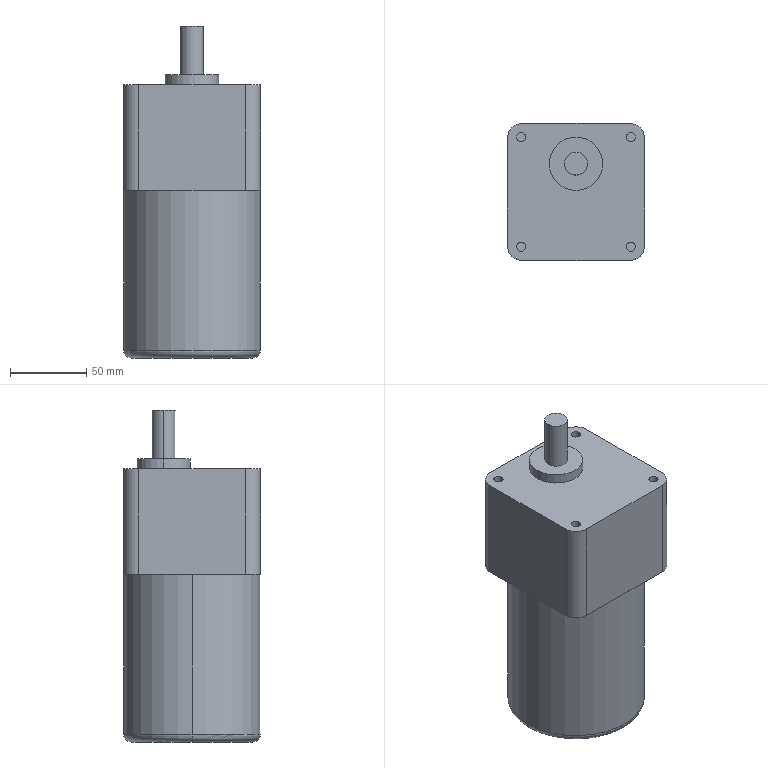Component | SolidWorks | --MA18S20041115GU-50KB90W-1 | 1 solid | 33 faces | box 90 x 90 x 218 mm | volume 1262403 mm3 | cylinder 18 | plane 13 | torus 2 | commonest cylinder face diameters 6 x8 20 x4 15 x2 35 x2 89.8 x2
build123d program:
from build123d import *

# Parameters (mm, degrees)
SKETCH1_W          = 90
SKETCH1_H          = 90
EXTRUDE1_DEPTH     = 69.5
SKETCH2_R          = 44.9
EXTRUDE2_DEPTH     = 110
SKETCH3_R          = 3
CUT_EXTRUDE1_DEPTH = 15
SKETCH4_R          = 17.5
EXTRUDE3_DEPTH     = 6.5
SKETCH5_R          = 7.5
EXTRUDE4_DEPTH     = 32
FILLET1_R          = 10
FILLET2_R          = 5


with BuildPart() as part:
    # Sketch1 → Extrude1 (new body)
    with BuildSketch(Plane.XY):
        Rectangle(SKETCH1_W, SKETCH1_H)
    extrude(amount=-EXTRUDE1_DEPTH)

    # Sketch2 → Extrude2 (add)
    with BuildSketch(Plane(origin=(0, 0, -69.5), x_dir=(-1, 0, 0), z_dir=(0, 0, -1))):
        with Locations(Location((0, 0, 0), (0, 0, 180))):
            Circle(SKETCH2_R)
    extrude(amount=EXTRUDE2_DEPTH)

    # Sketch3 → Cut-Extrude1 (cut)
    with BuildSketch(Plane.XY):
        with Locations((-36, 36)):
            Circle(SKETCH3_R)
        with Locations(Location((36, 36, 0), (0, 0, 180))):
            Circle(SKETCH3_R)
        with Locations((36, -36)):
            Circle(SKETCH3_R)
        with Locations(Location((-36, -36, 0), (0, 0, 180))):
            Circle(SKETCH3_R)
    extrude(amount=-CUT_EXTRUDE1_DEPTH, mode=Mode.SUBTRACT)

    # Sketch4 → Extrude3 (add)
    with BuildSketch(Plane.XY):
        with Locations(Location((0, 18.5, 0), (0, 0, 180))):
            Circle(SKETCH4_R)
    extrude(amount=EXTRUDE3_DEPTH)

    # Sketch5 → Extrude4 (add)
    with BuildSketch(Plane.XY.offset(6.5)):
        with Locations((0, 18.5)):
            Circle(SKETCH5_R)
    extrude(amount=EXTRUDE4_DEPTH)

    # Fillet1
    fillet1_edges = [part.edges().sort_by_distance(p)[0] for p in [
        (-45, 45, -34.75),
        (45, 45, -34.75),
        (45, -45, -34.75),
        (-45, -45, -34.75),
    ]]
    fillet(fillet1_edges, radius=FILLET1_R)

    # Fillet2
    fillet2_edges = [part.edges().sort_by_distance(p)[0] for p in [
        (-44.9, 0, -179.5),
    ]]
    fillet(fillet2_edges, radius=FILLET2_R)


solid = part.part

# Placed as in the assembly
solid = solid.moved(Location((245.885, -89.801, 61), (0, 0, 0)))
STEP:
#1=COLOUR_RGB('',0.7922,0.8196,0.9333);
#2=FILL_AREA_STYLE_COLOUR('',#1);
#3=FILL_AREA_STYLE('',(#2));
#4=SURFACE_STYLE_FILL_AREA(#3);
#5=SURFACE_SIDE_STYLE('',(#4));
#6=SURFACE_STYLE_USAGE(.BOTH.,#5);
#7=PRESENTATION_STYLE_ASSIGNMENT((#6));
#8=CARTESIAN_POINT('',(11.448,-3.535,-4.469));
#9=VERTEX_POINT('',#8);
#10=CARTESIAN_POINT('',(7.913,-3.535,-4.469));
#11=VERTEX_POINT('',#10);
#12=CARTESIAN_POINT('',(9.681,-3.535,-4.469));
#13=DIRECTION('',(0.,0.,1.));
#14=DIRECTION('',(-1.,0.,0.));
#15=AXIS2_PLACEMENT_3D('',#12,#13,#14);
#16=CIRCLE('',#15,1.768);
#17=EDGE_CURVE('',#9,#11,#16,.T.);
#18=ORIENTED_EDGE('',*,*,#17,.F.);
#19=CARTESIAN_POINT('',(11.251,-3.535,-4.665));
#20=VERTEX_POINT('',#19);
#21=CARTESIAN_POINT('',(11.251,-3.535,-4.469));
#22=DIRECTION('',(-0.,1.,0.));
#23=DIRECTION('',(-1.,0.,0.));
#24=AXIS2_PLACEMENT_3D('',#21,#22,#23);
#25=CIRCLE('',#24,0.1969);
#26=EDGE_CURVE('',#9,#20,#25,.T.);
#27=ORIENTED_EDGE('',*,*,#26,.T.);
#28=CARTESIAN_POINT('',(8.11,-3.535,-4.665));
#29=VERTEX_POINT('',#28);
#30=CARTESIAN_POINT('',(9.681,-3.535,-4.665));
#31=DIRECTION('',(0.,0.,-1.));
#32=DIRECTION('',(-1.,0.,0.));
#33=AXIS2_PLACEMENT_3D('',#30,#31,#32);
#34=CIRCLE('',#33,1.571);
#35=EDGE_CURVE('',#29,#20,#34,.T.);
#36=ORIENTED_EDGE('',*,*,#35,.F.);
#37=CARTESIAN_POINT('',(8.11,-3.535,-4.469));
#38=DIRECTION('',(0.,-1.,0.));
#39=DIRECTION('',(0.,0.,-1.));
#40=AXIS2_PLACEMENT_3D('',#37,#38,#39);
#41=CIRCLE('',#40,0.1969);
#42=EDGE_CURVE('',#11,#29,#41,.T.);
#43=ORIENTED_EDGE('',*,*,#42,.F.);
#44=EDGE_LOOP('',(#18,#27,#36,#43));
#45=FACE_OUTER_BOUND('',#44,.T.);
#46=CARTESIAN_POINT('',(9.681,-3.535,-4.469));
#47=DIRECTION('',(0.,0.,-1.));
#48=DIRECTION('',(-1.,0.,0.));
#49=AXIS2_PLACEMENT_3D('',#46,#47,#48);
#50=TOROIDAL_SURFACE('',#49,1.571,0.1969);
#51=ADVANCED_FACE('',(#45),#50,.T.);
#52=CARTESIAN_POINT('',(9.976,-2.807,3.917));
#53=VERTEX_POINT('',#52);
#54=CARTESIAN_POINT('',(9.385,-2.807,3.917));
#55=VERTEX_POINT('',#54);
#56=CARTESIAN_POINT('',(9.681,-2.807,3.917));
#57=DIRECTION('',(0.,0.,1.));
#58=DIRECTION('',(1.,0.,0.));
#59=AXIS2_PLACEMENT_3D('',#56,#57,#58);
#60=CIRCLE('',#59,0.2953);
#61=EDGE_CURVE('',#53,#55,#60,.T.);
#62=ORIENTED_EDGE('',*,*,#61,.F.);
#63=CARTESIAN_POINT('',(9.976,-2.807,2.657));
#64=VERTEX_POINT('',#63);
#65=CARTESIAN_POINT('',(9.976,-2.807,3.917));
#66=DIRECTION('',(0.,0.,-1.));
#67=VECTOR('',#66,39.37);
#68=LINE('',#65,#67);
#69=EDGE_CURVE('',#53,#64,#68,.T.);
#70=ORIENTED_EDGE('',*,*,#69,.T.);
#71=CARTESIAN_POINT('',(9.385,-2.807,2.657));
#72=VERTEX_POINT('',#71);
#73=CARTESIAN_POINT('',(9.681,-2.807,2.657));
#74=DIRECTION('',(0.,0.,1.));
#75=DIRECTION('',(1.,0.,0.));
#76=AXIS2_PLACEMENT_3D('',#73,#74,#75);
#77=CIRCLE('',#76,0.2953);
#78=EDGE_CURVE('',#64,#72,#77,.T.);
#79=ORIENTED_EDGE('',*,*,#78,.T.);
#80=CARTESIAN_POINT('',(9.385,-2.807,3.917));
#81=DIRECTION('',(0.,0.,-1.));
#82=VECTOR('',#81,39.37);
#83=LINE('',#80,#82);
#84=EDGE_CURVE('',#55,#72,#83,.T.);
#85=ORIENTED_EDGE('',*,*,#84,.F.);
#86=EDGE_LOOP('',(#62,#70,#79,#85));
#87=FACE_OUTER_BOUND('',#86,.T.);
#88=CARTESIAN_POINT('',(9.681,-2.807,3.917));
#89=DIRECTION('',(0.,0.,-1.));
#90=DIRECTION('',(-1.,0.,0.));
#91=AXIS2_PLACEMENT_3D('',#88,#89,#90);
#92=CYLINDRICAL_SURFACE('',#91,0.2953);
#93=ADVANCED_FACE('',(#87),#92,.T.);
#94=CARTESIAN_POINT('',(10.369,-2.807,2.657));
#95=VERTEX_POINT('',#94);
#96=CARTESIAN_POINT('',(8.992,-2.807,2.657));
#97=VERTEX_POINT('',#96);
#98=CARTESIAN_POINT('',(9.681,-2.807,2.657));
#99=DIRECTION('',(0.,0.,1.));
#100=DIRECTION('',(1.,0.,0.));
#101=AXIS2_PLACEMENT_3D('',#98,#99,#100);
#102=CIRCLE('',#101,0.689);
#103=EDGE_CURVE('',#95,#97,#102,.T.);
#104=ORIENTED_EDGE('',*,*,#103,.F.);
#105=CARTESIAN_POINT('',(10.369,-2.807,2.402));
#106=VERTEX_POINT('',#105);
#107=CARTESIAN_POINT('',(10.369,-2.807,2.657));
#108=DIRECTION('',(0.,0.,-1.));
#109=VECTOR('',#108,39.37);
#110=LINE('',#107,#109);
#111=EDGE_CURVE('',#95,#106,#110,.T.);
#112=ORIENTED_EDGE('',*,*,#111,.T.);
#113=CARTESIAN_POINT('',(8.992,-2.807,2.402));
#114=VERTEX_POINT('',#113);
#115=CARTESIAN_POINT('',(9.681,-2.807,2.402));
#116=DIRECTION('',(0.,0.,1.));
#117=DIRECTION('',(1.,0.,0.));
#118=AXIS2_PLACEMENT_3D('',#115,#116,#117);
#119=CIRCLE('',#118,0.689);
#120=EDGE_CURVE('',#106,#114,#119,.T.);
#121=ORIENTED_EDGE('',*,*,#120,.T.);
#122=CARTESIAN_POINT('',(8.992,-2.807,2.657));
#123=DIRECTION('',(0.,0.,-1.));
#124=VECTOR('',#123,39.37);
#125=LINE('',#122,#124);
#126=EDGE_CURVE('',#97,#114,#125,.T.);
#127=ORIENTED_EDGE('',*,*,#126,.F.);
#128=EDGE_LOOP('',(#104,#112,#121,#127));
#129=FACE_OUTER_BOUND('',#128,.T.);
#130=CARTESIAN_POINT('',(9.681,-2.807,2.657));
#131=DIRECTION('',(0.,0.,-1.));
#132=DIRECTION('',(-1.,0.,0.));
#133=AXIS2_PLACEMENT_3D('',#130,#131,#132);
#134=CYLINDRICAL_SURFACE('',#133,0.689);
#135=ADVANCED_FACE('',(#129),#134,.T.);
#136=CARTESIAN_POINT('',(8.145,-4.953,1.811));
#137=VERTEX_POINT('',#136);
#138=CARTESIAN_POINT('',(8.381,-4.953,1.811));
#139=VERTEX_POINT('',#138);
#140=CARTESIAN_POINT('',(8.263,-4.953,1.811));
#141=DIRECTION('',(0.,0.,1.));
#142=DIRECTION('',(-1.,0.,0.));
#143=AXIS2_PLACEMENT_3D('',#140,#141,#142);
#144=CIRCLE('',#143,0.1181);
#145=EDGE_CURVE('',#137,#139,#144,.T.);
#146=ORIENTED_EDGE('',*,*,#145,.F.);
#147=CARTESIAN_POINT('',(8.145,-4.953,2.402));
#148=VERTEX_POINT('',#147);
#149=CARTESIAN_POINT('',(8.145,-4.953,1.811));
#150=DIRECTION('',(0.,0.,1.));
#151=VECTOR('',#150,39.37);
#152=LINE('',#149,#151);
#153=EDGE_CURVE('',#137,#148,#152,.T.);
#154=ORIENTED_EDGE('',*,*,#153,.T.);
#155=CARTESIAN_POINT('',(8.381,-4.953,2.402));
#156=VERTEX_POINT('',#155);
#157=CARTESIAN_POINT('',(8.263,-4.953,2.402));
#158=DIRECTION('',(0.,0.,1.));
#159=DIRECTION('',(-1.,0.,0.));
#160=AXIS2_PLACEMENT_3D('',#157,#158,#159);
#161=CIRCLE('',#160,0.1181);
#162=EDGE_CURVE('',#148,#156,#161,.T.);
#163=ORIENTED_EDGE('',*,*,#162,.T.);
#164=CARTESIAN_POINT('',(8.381,-4.953,1.811));
#165=DIRECTION('',(0.,0.,1.));
#166=VECTOR('',#165,39.37);
#167=LINE('',#164,#166);
#168=EDGE_CURVE('',#139,#156,#167,.T.);
#169=ORIENTED_EDGE('',*,*,#168,.F.);
#170=EDGE_LOOP('',(#146,#154,#163,#169));
#171=FACE_OUTER_BOUND('',#170,.T.);
#172=CARTESIAN_POINT('',(8.263,-4.953,1.811));
#173=DIRECTION('',(0.,0.,1.));
#174=DIRECTION('',(1.,0.,0.));
#175=AXIS2_PLACEMENT_3D('',#172,#173,#174);
#176=CYLINDRICAL_SURFACE('',#175,0.1181);
#177=ADVANCED_FACE('',(#171),#176,.F.);
#178=CARTESIAN_POINT('',(10.98,-4.953,1.811));
#179=VERTEX_POINT('',#178);
#180=CARTESIAN_POINT('',(11.216,-4.953,1.811));
#181=VERTEX_POINT('',#180);
#182=CARTESIAN_POINT('',(11.098,-4.953,1.811));
#183=DIRECTION('',(0.,0.,1.));
#184=DIRECTION('',(1.,0.,0.));
#185=AXIS2_PLACEMENT_3D('',#182,#183,#184);
#186=CIRCLE('',#185,0.1181);
#187=EDGE_CURVE('',#179,#181,#186,.T.);
#188=ORIENTED_EDGE('',*,*,#187,.F.);
#189=CARTESIAN_POINT('',(10.98,-4.953,2.402));
#190=VERTEX_POINT('',#189);
#191=CARTESIAN_POINT('',(10.98,-4.953,1.811));
#192=DIRECTION('',(0.,0.,1.));
#193=VECTOR('',#192,39.37);
#194=LINE('',#191,#193);
#195=EDGE_CURVE('',#179,#190,#194,.T.);
#196=ORIENTED_EDGE('',*,*,#195,.T.);
#197=CARTESIAN_POINT('',(11.216,-4.953,2.402));
#198=VERTEX_POINT('',#197);
#199=CARTESIAN_POINT('',(11.098,-4.953,2.402));
#200=DIRECTION('',(0.,0.,1.));
#201=DIRECTION('',(1.,0.,0.));
#202=AXIS2_PLACEMENT_3D('',#199,#200,#201);
#203=CIRCLE('',#202,0.1181);
#204=EDGE_CURVE('',#190,#198,#203,.T.);
#205=ORIENTED_EDGE('',*,*,#204,.T.);
#206=CARTESIAN_POINT('',(11.216,-4.953,1.811));
#207=DIRECTION('',(0.,0.,1.));
#208=VECTOR('',#207,39.37);
#209=LINE('',#206,#208);
#210=EDGE_CURVE('',#181,#198,#209,.T.);
#211=ORIENTED_EDGE('',*,*,#210,.F.);
#212=EDGE_LOOP('',(#188,#196,#205,#211));
#213=FACE_OUTER_BOUND('',#212,.T.);
#214=CARTESIAN_POINT('',(11.098,-4.953,1.811));
#215=DIRECTION('',(0.,0.,1.));
#216=DIRECTION('',(1.,0.,0.));
#217=AXIS2_PLACEMENT_3D('',#214,#215,#216);
#218=CYLINDRICAL_SURFACE('',#217,0.1181);
#219=ADVANCED_FACE('',(#213),#218,.F.);
#220=CARTESIAN_POINT('',(10.98,-2.118,1.811));
#221=VERTEX_POINT('',#220);
#222=CARTESIAN_POINT('',(11.216,-2.118,1.811));
#223=VERTEX_POINT('',#222);
#224=CARTESIAN_POINT('',(11.098,-2.118,1.811));
#225=DIRECTION('',(0.,0.,1.));
#226=DIRECTION('',(-1.,0.,0.));
#227=AXIS2_PLACEMENT_3D('',#224,#225,#226);
#228=CIRCLE('',#227,0.1181);
#229=EDGE_CURVE('',#221,#223,#228,.T.);
#230=ORIENTED_EDGE('',*,*,#229,.F.);
#231=CARTESIAN_POINT('',(10.98,-2.118,2.402));
#232=VERTEX_POINT('',#231);
#233=CARTESIAN_POINT('',(10.98,-2.118,1.811));
#234=DIRECTION('',(0.,0.,1.));
#235=VECTOR('',#234,39.37);
#236=LINE('',#233,#235);
#237=EDGE_CURVE('',#221,#232,#236,.T.);
#238=ORIENTED_EDGE('',*,*,#237,.T.);
#239=CARTESIAN_POINT('',(11.216,-2.118,2.402));
#240=VERTEX_POINT('',#239);
#241=CARTESIAN_POINT('',(11.098,-2.118,2.402));
#242=DIRECTION('',(0.,0.,1.));
#243=DIRECTION('',(-1.,0.,0.));
#244=AXIS2_PLACEMENT_3D('',#241,#242,#243);
#245=CIRCLE('',#244,0.1181);
#246=EDGE_CURVE('',#232,#240,#245,.T.);
#247=ORIENTED_EDGE('',*,*,#246,.T.);
#248=CARTESIAN_POINT('',(11.216,-2.118,1.811));
#249=DIRECTION('',(0.,0.,1.));
#250=VECTOR('',#249,39.37);
#251=LINE('',#248,#250);
#252=EDGE_CURVE('',#223,#240,#251,.T.);
#253=ORIENTED_EDGE('',*,*,#252,.F.);
#254=EDGE_LOOP('',(#230,#238,#247,#253));
#255=FACE_OUTER_BOUND('',#254,.T.);
#256=CARTESIAN_POINT('',(11.098,-2.118,1.811));
#257=DIRECTION('',(0.,0.,1.));
#258=DIRECTION('',(1.,0.,0.));
#259=AXIS2_PLACEMENT_3D('',#256,#257,#258);
#260=CYLINDRICAL_SURFACE('',#259,0.1181);
#261=ADVANCED_FACE('',(#255),#260,.F.);
#262=CARTESIAN_POINT('',(8.145,-2.118,1.811));
#263=VERTEX_POINT('',#262);
#264=CARTESIAN_POINT('',(8.381,-2.118,1.811));
#265=VERTEX_POINT('',#264);
#266=CARTESIAN_POINT('',(8.263,-2.118,1.811));
#267=DIRECTION('',(0.,0.,1.));
#268=DIRECTION('',(1.,0.,0.));
#269=AXIS2_PLACEMENT_3D('',#266,#267,#268);
#270=CIRCLE('',#269,0.1181);
#271=EDGE_CURVE('',#263,#265,#270,.T.);
#272=ORIENTED_EDGE('',*,*,#271,.F.);
#273=CARTESIAN_POINT('',(8.145,-2.118,2.402));
#274=VERTEX_POINT('',#273);
#275=CARTESIAN_POINT('',(8.145,-2.118,1.811));
#276=DIRECTION('',(0.,0.,1.));
#277=VECTOR('',#276,39.37);
#278=LINE('',#275,#277);
#279=EDGE_CURVE('',#263,#274,#278,.T.);
#280=ORIENTED_EDGE('',*,*,#279,.T.);
#281=CARTESIAN_POINT('',(8.381,-2.118,2.402));
#282=VERTEX_POINT('',#281);
#283=CARTESIAN_POINT('',(8.263,-2.118,2.402));
#284=DIRECTION('',(0.,0.,1.));
#285=DIRECTION('',(1.,0.,0.));
#286=AXIS2_PLACEMENT_3D('',#283,#284,#285);
#287=CIRCLE('',#286,0.1181);
#288=EDGE_CURVE('',#274,#282,#287,.T.);
#289=ORIENTED_EDGE('',*,*,#288,.T.);
#290=CARTESIAN_POINT('',(8.381,-2.118,1.811));
#291=DIRECTION('',(0.,0.,1.));
#292=VECTOR('',#291,39.37);
#293=LINE('',#290,#292);
#294=EDGE_CURVE('',#265,#282,#293,.T.);
#295=ORIENTED_EDGE('',*,*,#294,.F.);
#296=EDGE_LOOP('',(#272,#280,#289,#295));
#297=FACE_OUTER_BOUND('',#296,.T.);
#298=CARTESIAN_POINT('',(8.263,-2.118,1.811));
#299=DIRECTION('',(0.,0.,1.));
#300=DIRECTION('',(1.,0.,0.));
#301=AXIS2_PLACEMENT_3D('',#298,#299,#300);
#302=CYLINDRICAL_SURFACE('',#301,0.1181);
#303=ADVANCED_FACE('',(#297),#302,.F.);
#304=ORIENTED_EDGE('',*,*,#17,.T.);
#305=CARTESIAN_POINT('',(7.913,-3.535,-0.3346));
#306=VERTEX_POINT('',#305);
#307=CARTESIAN_POINT('',(7.913,-3.535,-4.665));
#308=DIRECTION('',(0.,0.,1.));
#309=VECTOR('',#308,39.37);
#310=LINE('',#307,#309);
#311=EDGE_CURVE('',#11,#306,#310,.T.);
#312=ORIENTED_EDGE('',*,*,#311,.T.);
#313=CARTESIAN_POINT('',(11.448,-3.535,-0.3346));
#314=VERTEX_POINT('',#313);
#315=CARTESIAN_POINT('',(9.681,-3.535,-0.3346));
#316=DIRECTION('',(0.,0.,-1.));
#317=DIRECTION('',(1.,0.,0.));
#318=AXIS2_PLACEMENT_3D('',#315,#316,#317);
#319=CIRCLE('',#318,1.768);
#320=EDGE_CURVE('',#306,#314,#319,.T.);
#321=ORIENTED_EDGE('',*,*,#320,.T.);
#322=CARTESIAN_POINT('',(11.448,-3.535,-4.665));
#323=DIRECTION('',(0.,0.,1.));
#324=VECTOR('',#323,39.37);
#325=LINE('',#322,#324);
#326=EDGE_CURVE('',#9,#314,#325,.T.);
#327=ORIENTED_EDGE('',*,*,#326,.F.);
#328=EDGE_LOOP('',(#304,#312,#321,#327));
#329=FACE_OUTER_BOUND('',#328,.T.);
#330=CARTESIAN_POINT('',(9.681,-3.535,-4.665));
#331=DIRECTION('',(0.,0.,1.));
#332=DIRECTION('',(1.,0.,0.));
#333=AXIS2_PLACEMENT_3D('',#330,#331,#332);
#334=CYLINDRICAL_SURFACE('',#333,1.768);
#335=ADVANCED_FACE('',(#329),#334,.T.);
#336=CARTESIAN_POINT('',(9.681,-2.807,2.657));
#337=DIRECTION('',(0.,0.,1.));
#338=DIRECTION('',(1.,0.,0.));
#339=AXIS2_PLACEMENT_3D('',#336,#337,#338);
#340=CIRCLE('',#339,0.689);
#341=EDGE_CURVE('',#97,#95,#340,.T.);
#342=ORIENTED_EDGE('',*,*,#341,.T.);
#343=ORIENTED_EDGE('',*,*,#103,.T.);
#344=EDGE_LOOP('',(#342,#343));
#345=FACE_OUTER_BOUND('',#344,.T.);
#346=CARTESIAN_POINT('',(9.681,-2.807,2.657));
#347=DIRECTION('',(0.,0.,1.));
#348=DIRECTION('',(1.,0.,0.));
#349=AXIS2_PLACEMENT_3D('',#346,#347,#348);
#350=CIRCLE('',#349,0.2953);
#351=EDGE_CURVE('',#72,#64,#350,.T.);
#352=ORIENTED_EDGE('',*,*,#351,.F.);
#353=ORIENTED_EDGE('',*,*,#78,.F.);
#354=EDGE_LOOP('',(#352,#353));
#355=FACE_BOUND('',#354,.T.);
#356=CARTESIAN_POINT('',(9.681,-2.807,2.657));
#357=DIRECTION('',(0.,0.,1.));
#358=DIRECTION('',(1.,0.,0.));
#359=AXIS2_PLACEMENT_3D('',#356,#357,#358);
#360=PLANE('',#359);
#361=ADVANCED_FACE('',(#345,#355),#360,.T.);
#362=CARTESIAN_POINT('',(7.909,-2.158,2.402));
#363=VERTEX_POINT('',#362);
#364=CARTESIAN_POINT('',(7.909,-4.913,2.402));
#365=VERTEX_POINT('',#364);
#366=CARTESIAN_POINT('',(7.909,-1.764,2.402));
#367=DIRECTION('',(0.,-1.,0.));
#368=VECTOR('',#367,39.37);
#369=LINE('',#366,#368);
#370=EDGE_CURVE('',#363,#365,#369,.T.);
#371=ORIENTED_EDGE('',*,*,#370,.T.);
#372=CARTESIAN_POINT('',(8.303,-5.307,2.402));
#373=VERTEX_POINT('',#372);
#374=CARTESIAN_POINT('',(8.303,-4.913,2.402));
#375=DIRECTION('',(0.,0.,1.));
#376=DIRECTION('',(1.,0.,0.));
#377=AXIS2_PLACEMENT_3D('',#374,#375,#376);
#378=CIRCLE('',#377,0.3937);
#379=EDGE_CURVE('',#365,#373,#378,.T.);
#380=ORIENTED_EDGE('',*,*,#379,.T.);
#381=CARTESIAN_POINT('',(11.058,-5.307,2.402));
#382=VERTEX_POINT('',#381);
#383=CARTESIAN_POINT('',(7.909,-5.307,2.402));
#384=DIRECTION('',(1.,0.,0.));
#385=VECTOR('',#384,39.37);
#386=LINE('',#383,#385);
#387=EDGE_CURVE('',#373,#382,#386,.T.);
#388=ORIENTED_EDGE('',*,*,#387,.T.);
#389=CARTESIAN_POINT('',(11.452,-4.913,2.402));
#390=VERTEX_POINT('',#389);
#391=CARTESIAN_POINT('',(11.058,-4.913,2.402));
#392=DIRECTION('',(0.,0.,1.));
#393=DIRECTION('',(1.,0.,0.));
#394=AXIS2_PLACEMENT_3D('',#391,#392,#393);
#395=CIRCLE('',#394,0.3937);
#396=EDGE_CURVE('',#382,#390,#395,.T.);
#397=ORIENTED_EDGE('',*,*,#396,.T.);
#398=CARTESIAN_POINT('',(11.452,-2.158,2.402));
#399=VERTEX_POINT('',#398);
#400=CARTESIAN_POINT('',(11.452,-1.764,2.402));
#401=DIRECTION('',(-0.,1.,0.));
#402=VECTOR('',#401,39.37);
#403=LINE('',#400,#402);
#404=EDGE_CURVE('',#390,#399,#403,.T.);
#405=ORIENTED_EDGE('',*,*,#404,.T.);
#406=CARTESIAN_POINT('',(11.058,-1.764,2.402));
#407=VERTEX_POINT('',#406);
#408=CARTESIAN_POINT('',(11.058,-2.158,2.402));
#409=DIRECTION('',(0.,0.,1.));
#410=DIRECTION('',(1.,0.,0.));
#411=AXIS2_PLACEMENT_3D('',#408,#409,#410);
#412=CIRCLE('',#411,0.3937);
#413=EDGE_CURVE('',#399,#407,#412,.T.);
#414=ORIENTED_EDGE('',*,*,#413,.T.);
#415=CARTESIAN_POINT('',(8.303,-1.764,2.402));
#416=VERTEX_POINT('',#415);
#417=CARTESIAN_POINT('',(7.909,-1.764,2.402));
#418=DIRECTION('',(-1.,-0.,0.));
#419=VECTOR('',#418,39.37);
#420=LINE('',#417,#419);
#421=EDGE_CURVE('',#407,#416,#420,.T.);
#422=ORIENTED_EDGE('',*,*,#421,.T.);
#423=CARTESIAN_POINT('',(8.303,-2.158,2.402));
#424=DIRECTION('',(0.,0.,1.));
#425=DIRECTION('',(1.,0.,0.));
#426=AXIS2_PLACEMENT_3D('',#423,#424,#425);
#427=CIRCLE('',#426,0.3937);
#428=EDGE_CURVE('',#416,#363,#427,.T.);
#429=ORIENTED_EDGE('',*,*,#428,.T.);
#430=EDGE_LOOP('',(#371,#380,#388,#397,#405,#414,#422,#429));
#431=FACE_OUTER_BOUND('',#430,.T.);
#432=CARTESIAN_POINT('',(8.263,-2.118,2.402));
#433=DIRECTION('',(0.,0.,1.));
#434=DIRECTION('',(1.,0.,0.));
#435=AXIS2_PLACEMENT_3D('',#432,#433,#434);
#436=CIRCLE('',#435,0.1181);
#437=EDGE_CURVE('',#282,#274,#436,.T.);
#438=ORIENTED_EDGE('',*,*,#437,.F.);
#439=ORIENTED_EDGE('',*,*,#288,.F.);
#440=EDGE_LOOP('',(#438,#439));
#441=FACE_BOUND('',#440,.T.);
#442=CARTESIAN_POINT('',(11.098,-2.118,2.402));
#443=DIRECTION('',(0.,0.,1.));
#444=DIRECTION('',(-1.,0.,0.));
#445=AXIS2_PLACEMENT_3D('',#442,#443,#444);
#446=CIRCLE('',#445,0.1181);
#447=EDGE_CURVE('',#240,#232,#446,.T.);
#448=ORIENTED_EDGE('',*,*,#447,.F.);
#449=ORIENTED_EDGE('',*,*,#246,.F.);
#450=EDGE_LOOP('',(#448,#449));
#451=FACE_BOUND('',#450,.T.);
#452=CARTESIAN_POINT('',(11.098,-4.953,2.402));
#453=DIRECTION('',(0.,0.,1.));
#454=DIRECTION('',(1.,0.,0.));
#455=AXIS2_PLACEMENT_3D('',#452,#453,#454);
#456=CIRCLE('',#455,0.1181);
#457=EDGE_CURVE('',#198,#190,#456,.T.);
#458=ORIENTED_EDGE('',*,*,#457,.F.);
#459=ORIENTED_EDGE('',*,*,#204,.F.);
#460=EDGE_LOOP('',(#458,#459));
#461=FACE_BOUND('',#460,.T.);
#462=CARTESIAN_POINT('',(8.263,-4.953,2.402));
#463=DIRECTION('',(0.,0.,1.));
#464=DIRECTION('',(-1.,0.,0.));
#465=AXIS2_PLACEMENT_3D('',#462,#463,#464);
#466=CIRCLE('',#465,0.1181);
#467=EDGE_CURVE('',#156,#148,#466,.T.);
#468=ORIENTED_EDGE('',*,*,#467,.F.);
#469=ORIENTED_EDGE('',*,*,#162,.F.);
#470=EDGE_LOOP('',(#468,#469));
#471=FACE_BOUND('',#470,.T.);
#472=CARTESIAN_POINT('',(9.681,-2.807,2.402));
#473=DIRECTION('',(0.,0.,1.));
#474=DIRECTION('',(1.,0.,0.));
#475=AXIS2_PLACEMENT_3D('',#472,#473,#474);
#476=CIRCLE('',#475,0.689);
#477=EDGE_CURVE('',#114,#106,#476,.T.);
#478=ORIENTED_EDGE('',*,*,#477,.F.);
#479=ORIENTED_EDGE('',*,*,#120,.F.);
#480=EDGE_LOOP('',(#478,#479));
#481=FACE_BOUND('',#480,.T.);
#482=CARTESIAN_POINT('',(7.909,-5.307,2.402));
#483=DIRECTION('',(0.,0.,1.));
#484=DIRECTION('',(1.,0.,0.));
#485=AXIS2_PLACEMENT_3D('',#482,#483,#484);
#486=PLANE('',#485);
#487=ADVANCED_FACE('',(#431,#441,#451,#461,#471,#481),#486,.T.);
#488=CARTESIAN_POINT('',(8.303,-5.307,-0.3346));
#489=VERTEX_POINT('',#488);
#490=CARTESIAN_POINT('',(11.058,-5.307,-0.3346));
#491=VERTEX_POINT('',#490);
#492=CARTESIAN_POINT('',(7.909,-5.307,-0.3346));
#493=DIRECTION('',(1.,0.,0.));
#494=VECTOR('',#493,39.37);
#495=LINE('',#492,#494);
#496=EDGE_CURVE('',#489,#491,#495,.T.);
#497=ORIENTED_EDGE('',*,*,#496,.F.);
#498=CARTESIAN_POINT('',(7.909,-4.913,-0.3346));
#499=VERTEX_POINT('',#498);
#500=CARTESIAN_POINT('',(8.303,-4.913,-0.3346));
#501=DIRECTION('',(0.,0.,-1.));
#502=DIRECTION('',(1.,0.,0.));
#503=AXIS2_PLACEMENT_3D('',#500,#501,#502);
#504=CIRCLE('',#503,0.3937);
#505=EDGE_CURVE('',#489,#499,#504,.T.);
#506=ORIENTED_EDGE('',*,*,#505,.T.);
#507=CARTESIAN_POINT('',(7.909,-2.158,-0.3346));
#508=VERTEX_POINT('',#507);
#509=CARTESIAN_POINT('',(7.909,-1.764,-0.3346));
#510=DIRECTION('',(0.,-1.,0.));
#511=VECTOR('',#510,39.37);
#512=LINE('',#509,#511);
#513=EDGE_CURVE('',#508,#499,#512,.T.);
#514=ORIENTED_EDGE('',*,*,#513,.F.);
#515=CARTESIAN_POINT('',(8.303,-1.764,-0.3346));
#516=VERTEX_POINT('',#515);
#517=CARTESIAN_POINT('',(8.303,-2.158,-0.3346));
#518=DIRECTION('',(0.,0.,-1.));
#519=DIRECTION('',(1.,0.,0.));
#520=AXIS2_PLACEMENT_3D('',#517,#518,#519);
#521=CIRCLE('',#520,0.3937);
#522=EDGE_CURVE('',#508,#516,#521,.T.);
#523=ORIENTED_EDGE('',*,*,#522,.T.);
#524=CARTESIAN_POINT('',(11.058,-1.764,-0.3346));
#525=VERTEX_POINT('',#524);
#526=CARTESIAN_POINT('',(7.909,-1.764,-0.3346));
#527=DIRECTION('',(-1.,-0.,0.));
#528=VECTOR('',#527,39.37);
#529=LINE('',#526,#528);
#530=EDGE_CURVE('',#525,#516,#529,.T.);
#531=ORIENTED_EDGE('',*,*,#530,.F.);
#532=CARTESIAN_POINT('',(11.452,-2.158,-0.3346));
#533=VERTEX_POINT('',#532);
#534=CARTESIAN_POINT('',(11.058,-2.158,-0.3346));
#535=DIRECTION('',(0.,0.,-1.));
#536=DIRECTION('',(1.,0.,0.));
#537=AXIS2_PLACEMENT_3D('',#534,#535,#536);
#538=CIRCLE('',#537,0.3937);
#539=EDGE_CURVE('',#525,#533,#538,.T.);
#540=ORIENTED_EDGE('',*,*,#539,.T.);
#541=CARTESIAN_POINT('',(11.452,-4.913,-0.3346));
#542=VERTEX_POINT('',#541);
#543=CARTESIAN_POINT('',(11.452,-1.764,-0.3346));
#544=DIRECTION('',(-0.,1.,0.));
#545=VECTOR('',#544,39.37);
#546=LINE('',#543,#545);
#547=EDGE_CURVE('',#542,#533,#546,.T.);
#548=ORIENTED_EDGE('',*,*,#547,.F.);
#549=CARTESIAN_POINT('',(11.058,-4.913,-0.3346));
#550=DIRECTION('',(0.,0.,-1.));
#551=DIRECTION('',(1.,0.,0.));
#552=AXIS2_PLACEMENT_3D('',#549,#550,#551);
#553=CIRCLE('',#552,0.3937);
#554=EDGE_CURVE('',#542,#491,#553,.T.);
#555=ORIENTED_EDGE('',*,*,#554,.T.);
#556=EDGE_LOOP('',(#497,#506,#514,#523,#531,#540,#548,#555));
#557=FACE_OUTER_BOUND('',#556,.T.);
#558=CARTESIAN_POINT('',(9.681,-3.535,-0.3346));
#559=DIRECTION('',(0.,0.,-1.));
#560=DIRECTION('',(1.,0.,0.));
#561=AXIS2_PLACEMENT_3D('',#558,#559,#560);
#562=CIRCLE('',#561,1.768);
#563=EDGE_CURVE('',#314,#306,#562,.T.);
#564=ORIENTED_EDGE('',*,*,#563,.F.);
#565=ORIENTED_EDGE('',*,*,#320,.F.);
#566=EDGE_LOOP('',(#564,#565));
#567=FACE_BOUND('',#566,.T.);
#568=CARTESIAN_POINT('',(7.909,-5.307,-0.3346));
#569=DIRECTION('',(0.,0.,1.));
#570=DIRECTION('',(1.,0.,0.));
#571=AXIS2_PLACEMENT_3D('',#568,#569,#570);
#572=PLANE('',#571);
#573=ADVANCED_FACE('',(#557,#567),#572,.F.);
#574=ORIENTED_EDGE('',*,*,#513,.T.);
#575=CARTESIAN_POINT('',(7.909,-4.913,-0.3346));
#576=DIRECTION('',(0.,0.,1.));
#577=VECTOR('',#576,39.37);
#578=LINE('',#575,#577);
#579=EDGE_CURVE('',#499,#365,#578,.T.);
#580=ORIENTED_EDGE('',*,*,#579,.T.);
#581=ORIENTED_EDGE('',*,*,#370,.F.);
#582=CARTESIAN_POINT('',(7.909,-2.158,-0.3346));
#583=DIRECTION('',(0.,0.,-1.));
#584=VECTOR('',#583,39.37);
#585=LINE('',#582,#584);
#586=EDGE_CURVE('',#363,#508,#585,.T.);
#587=ORIENTED_EDGE('',*,*,#586,.T.);
#588=EDGE_LOOP('',(#574,#580,#581,#587));
#589=FACE_OUTER_BOUND('',#588,.T.);
#590=CARTESIAN_POINT('',(7.909,-1.764,-0.3346));
#591=DIRECTION('',(-1.,-0.,0.));
#592=DIRECTION('',(0.,-1.,0.));
#593=AXIS2_PLACEMENT_3D('',#590,#591,#592);
#594=PLANE('',#593);
#595=ADVANCED_FACE('',(#589),#594,.T.);
#596=ORIENTED_EDGE('',*,*,#530,.T.);
#597=CARTESIAN_POINT('',(8.303,-1.764,-0.3346));
#598=DIRECTION('',(0.,0.,1.));
#599=VECTOR('',#598,39.37);
#600=LINE('',#597,#599);
#601=EDGE_CURVE('',#516,#416,#600,.T.);
#602=ORIENTED_EDGE('',*,*,#601,.T.);
#603=ORIENTED_EDGE('',*,*,#421,.F.);
#604=CARTESIAN_POINT('',(11.058,-1.764,-0.3346));
#605=DIRECTION('',(0.,0.,-1.));
#606=VECTOR('',#605,39.37);
#607=LINE('',#604,#606);
#608=EDGE_CURVE('',#407,#525,#607,.T.);
#609=ORIENTED_EDGE('',*,*,#608,.T.);
#610=EDGE_LOOP('',(#596,#602,#603,#609));
#611=FACE_OUTER_BOUND('',#610,.T.);
#612=CARTESIAN_POINT('',(7.909,-1.764,-0.3346));
#613=DIRECTION('',(-0.,1.,0.));
#614=DIRECTION('',(-1.,-0.,0.));
#615=AXIS2_PLACEMENT_3D('',#612,#613,#614);
#616=PLANE('',#615);
#617=ADVANCED_FACE('',(#611),#616,.T.);
#618=ORIENTED_EDGE('',*,*,#404,.F.);
#619=CARTESIAN_POINT('',(11.452,-4.913,-0.3346));
#620=DIRECTION('',(0.,0.,-1.));
#621=VECTOR('',#620,39.37);
#622=LINE('',#619,#621);
#623=EDGE_CURVE('',#390,#542,#622,.T.);
#624=ORIENTED_EDGE('',*,*,#623,.T.);
#625=ORIENTED_EDGE('',*,*,#547,.T.);
#626=CARTESIAN_POINT('',(11.452,-2.158,-0.3346));
#627=DIRECTION('',(0.,0.,1.));
#628=VECTOR('',#627,39.37);
#629=LINE('',#626,#628);
#630=EDGE_CURVE('',#533,#399,#629,.T.);
#631=ORIENTED_EDGE('',*,*,#630,.T.);
#632=EDGE_LOOP('',(#618,#624,#625,#631));
#633=FACE_OUTER_BOUND('',#632,.T.);
#634=CARTESIAN_POINT('',(11.452,-1.764,-0.3346));
#635=DIRECTION('',(1.,0.,0.));
#636=DIRECTION('',(-0.,1.,0.));
#637=AXIS2_PLACEMENT_3D('',#634,#635,#636);
#638=PLANE('',#637);
#639=ADVANCED_FACE('',(#633),#638,.T.);
#640=ORIENTED_EDGE('',*,*,#387,.F.);
#641=CARTESIAN_POINT('',(8.303,-5.307,-0.3346));
#642=DIRECTION('',(0.,0.,-1.));
#643=VECTOR('',#642,39.37);
#644=LINE('',#641,#643);
#645=EDGE_CURVE('',#373,#489,#644,.T.);
#646=ORIENTED_EDGE('',*,*,#645,.T.);
#647=ORIENTED_EDGE('',*,*,#496,.T.);
#648=CARTESIAN_POINT('',(11.058,-5.307,-0.3346));
#649=DIRECTION('',(0.,0.,1.));
#650=VECTOR('',#649,39.37);
#651=LINE('',#648,#650);
#652=EDGE_CURVE('',#491,#382,#651,.T.);
#653=ORIENTED_EDGE('',*,*,#652,.T.);
#654=EDGE_LOOP('',(#640,#646,#647,#653));
#655=FACE_OUTER_BOUND('',#654,.T.);
#656=CARTESIAN_POINT('',(7.909,-5.307,-0.3346));
#657=DIRECTION('',(0.,-1.,0.));
#658=DIRECTION('',(1.,0.,0.));
#659=AXIS2_PLACEMENT_3D('',#656,#657,#658);
#660=PLANE('',#659);
#661=ADVANCED_FACE('',(#655),#660,.T.);
#662=ORIENTED_EDGE('',*,*,#311,.F.);
#663=CARTESIAN_POINT('',(9.681,-3.535,-4.469));
#664=DIRECTION('',(0.,0.,1.));
#665=DIRECTION('',(-1.,0.,0.));
#666=AXIS2_PLACEMENT_3D('',#663,#664,#665);
#667=CIRCLE('',#666,1.768);
#668=EDGE_CURVE('',#11,#9,#667,.T.);
#669=ORIENTED_EDGE('',*,*,#668,.T.);
#670=ORIENTED_EDGE('',*,*,#326,.T.);
#671=ORIENTED_EDGE('',*,*,#563,.T.);
#672=EDGE_LOOP('',(#662,#669,#670,#671));
#673=FACE_OUTER_BOUND('',#672,.T.);
#674=CARTESIAN_POINT('',(9.681,-3.535,-4.665));
#675=DIRECTION('',(0.,0.,1.));
#676=DIRECTION('',(1.,0.,0.));
#677=AXIS2_PLACEMENT_3D('',#674,#675,#676);
#678=CYLINDRICAL_SURFACE('',#677,1.768);
#679=ADVANCED_FACE('',(#673),#678,.T.);
#680=ORIENTED_EDGE('',*,*,#35,.T.);
#681=CARTESIAN_POINT('',(9.681,-3.535,-4.665));
#682=DIRECTION('',(0.,0.,-1.));
#683=DIRECTION('',(-1.,0.,0.));
#684=AXIS2_PLACEMENT_3D('',#681,#682,#683);
#685=CIRCLE('',#684,1.571);
#686=EDGE_CURVE('',#20,#29,#685,.T.);
#687=ORIENTED_EDGE('',*,*,#686,.T.);
#688=EDGE_LOOP('',(#680,#687));
#689=FACE_OUTER_BOUND('',#688,.T.);
#690=CARTESIAN_POINT('',(9.681,-3.535,-4.665));
#691=DIRECTION('',(0.,0.,-1.));
#692=DIRECTION('',(-1.,0.,0.));
#693=AXIS2_PLACEMENT_3D('',#690,#691,#692);
#694=PLANE('',#693);
#695=ADVANCED_FACE('',(#689),#694,.T.);
#696=ORIENTED_EDGE('',*,*,#279,.F.);
#697=CARTESIAN_POINT('',(8.263,-2.118,1.811));
#698=DIRECTION('',(0.,0.,1.));
#699=DIRECTION('',(1.,0.,0.));
#700=AXIS2_PLACEMENT_3D('',#697,#698,#699);
#701=CIRCLE('',#700,0.1181);
#702=EDGE_CURVE('',#265,#263,#701,.T.);
#703=ORIENTED_EDGE('',*,*,#702,.F.);
#704=ORIENTED_EDGE('',*,*,#294,.T.);
#705=ORIENTED_EDGE('',*,*,#437,.T.);
#706=EDGE_LOOP('',(#696,#703,#704,#705));
#707=FACE_OUTER_BOUND('',#706,.T.);
#708=CARTESIAN_POINT('',(8.263,-2.118,1.811));
#709=DIRECTION('',(0.,0.,1.));
#710=DIRECTION('',(1.,0.,0.));
#711=AXIS2_PLACEMENT_3D('',#708,#709,#710);
#712=CYLINDRICAL_SURFACE('',#711,0.1181);
#713=ADVANCED_FACE('',(#707),#712,.F.);
#714=ORIENTED_EDGE('',*,*,#702,.T.);
#715=ORIENTED_EDGE('',*,*,#271,.T.);
#716=EDGE_LOOP('',(#714,#715));
#717=FACE_OUTER_BOUND('',#716,.T.);
#718=CARTESIAN_POINT('',(8.263,-2.118,1.811));
#719=DIRECTION('',(0.,0.,1.));
#720=DIRECTION('',(1.,0.,0.));
#721=AXIS2_PLACEMENT_3D('',#718,#719,#720);
#722=PLANE('',#721);
#723=ADVANCED_FACE('',(#717),#722,.T.);
#724=ORIENTED_EDGE('',*,*,#237,.F.);
#725=CARTESIAN_POINT('',(11.098,-2.118,1.811));
#726=DIRECTION('',(0.,0.,1.));
#727=DIRECTION('',(-1.,0.,0.));
#728=AXIS2_PLACEMENT_3D('',#725,#726,#727);
#729=CIRCLE('',#728,0.1181);
#730=EDGE_CURVE('',#223,#221,#729,.T.);
#731=ORIENTED_EDGE('',*,*,#730,.F.);
#732=ORIENTED_EDGE('',*,*,#252,.T.);
#733=ORIENTED_EDGE('',*,*,#447,.T.);
#734=EDGE_LOOP('',(#724,#731,#732,#733));
#735=FACE_OUTER_BOUND('',#734,.T.);
#736=CARTESIAN_POINT('',(11.098,-2.118,1.811));
#737=DIRECTION('',(0.,0.,1.));
#738=DIRECTION('',(1.,0.,0.));
#739=AXIS2_PLACEMENT_3D('',#736,#737,#738);
#740=CYLINDRICAL_SURFACE('',#739,0.1181);
#741=ADVANCED_FACE('',(#735),#740,.F.);
#742=ORIENTED_EDGE('',*,*,#730,.T.);
#743=ORIENTED_EDGE('',*,*,#229,.T.);
#744=EDGE_LOOP('',(#742,#743));
#745=FACE_OUTER_BOUND('',#744,.T.);
#746=CARTESIAN_POINT('',(11.098,-2.118,1.811));
#747=DIRECTION('',(0.,0.,-1.));
#748=DIRECTION('',(-1.,0.,0.));
#749=AXIS2_PLACEMENT_3D('',#746,#747,#748);
#750=PLANE('',#749);
#751=ADVANCED_FACE('',(#745),#750,.F.);
#752=ORIENTED_EDGE('',*,*,#195,.F.);
#753=CARTESIAN_POINT('',(11.098,-4.953,1.811));
#754=DIRECTION('',(0.,0.,1.));
#755=DIRECTION('',(1.,0.,0.));
#756=AXIS2_PLACEMENT_3D('',#753,#754,#755);
#757=CIRCLE('',#756,0.1181);
#758=EDGE_CURVE('',#181,#179,#757,.T.);
#759=ORIENTED_EDGE('',*,*,#758,.F.);
#760=ORIENTED_EDGE('',*,*,#210,.T.);
#761=ORIENTED_EDGE('',*,*,#457,.T.);
#762=EDGE_LOOP('',(#752,#759,#760,#761));
#763=FACE_OUTER_BOUND('',#762,.T.);
#764=CARTESIAN_POINT('',(11.098,-4.953,1.811));
#765=DIRECTION('',(0.,0.,1.));
#766=DIRECTION('',(1.,0.,0.));
#767=AXIS2_PLACEMENT_3D('',#764,#765,#766);
#768=CYLINDRICAL_SURFACE('',#767,0.1181);
#769=ADVANCED_FACE('',(#763),#768,.F.);
#770=ORIENTED_EDGE('',*,*,#758,.T.);
#771=ORIENTED_EDGE('',*,*,#187,.T.);
#772=EDGE_LOOP('',(#770,#771));
#773=FACE_OUTER_BOUND('',#772,.T.);
#774=CARTESIAN_POINT('',(11.098,-4.953,1.811));
#775=DIRECTION('',(0.,0.,1.));
#776=DIRECTION('',(1.,0.,0.));
#777=AXIS2_PLACEMENT_3D('',#774,#775,#776);
#778=PLANE('',#777);
#779=ADVANCED_FACE('',(#773),#778,.T.);
#780=ORIENTED_EDGE('',*,*,#153,.F.);
#781=CARTESIAN_POINT('',(8.263,-4.953,1.811));
#782=DIRECTION('',(0.,0.,1.));
#783=DIRECTION('',(-1.,0.,0.));
#784=AXIS2_PLACEMENT_3D('',#781,#782,#783);
#785=CIRCLE('',#784,0.1181);
#786=EDGE_CURVE('',#139,#137,#785,.T.);
#787=ORIENTED_EDGE('',*,*,#786,.F.);
#788=ORIENTED_EDGE('',*,*,#168,.T.);
#789=ORIENTED_EDGE('',*,*,#467,.T.);
#790=EDGE_LOOP('',(#780,#787,#788,#789));
#791=FACE_OUTER_BOUND('',#790,.T.);
#792=CARTESIAN_POINT('',(8.263,-4.953,1.811));
#793=DIRECTION('',(0.,0.,1.));
#794=DIRECTION('',(1.,0.,0.));
#795=AXIS2_PLACEMENT_3D('',#792,#793,#794);
#796=CYLINDRICAL_SURFACE('',#795,0.1181);
#797=ADVANCED_FACE('',(#791),#796,.F.);
#798=ORIENTED_EDGE('',*,*,#786,.T.);
#799=ORIENTED_EDGE('',*,*,#145,.T.);
#800=EDGE_LOOP('',(#798,#799));
#801=FACE_OUTER_BOUND('',#800,.T.);
#802=CARTESIAN_POINT('',(8.263,-4.953,1.811));
#803=DIRECTION('',(0.,0.,-1.));
#804=DIRECTION('',(-1.,0.,0.));
#805=AXIS2_PLACEMENT_3D('',#802,#803,#804);
#806=PLANE('',#805);
#807=ADVANCED_FACE('',(#801),#806,.F.);
#808=ORIENTED_EDGE('',*,*,#111,.F.);
#809=ORIENTED_EDGE('',*,*,#341,.F.);
#810=ORIENTED_EDGE('',*,*,#126,.T.);
#811=ORIENTED_EDGE('',*,*,#477,.T.);
#812=EDGE_LOOP('',(#808,#809,#810,#811));
#813=FACE_OUTER_BOUND('',#812,.T.);
#814=CARTESIAN_POINT('',(9.681,-2.807,2.657));
#815=DIRECTION('',(0.,0.,-1.));
#816=DIRECTION('',(-1.,0.,0.));
#817=AXIS2_PLACEMENT_3D('',#814,#815,#816);
#818=CYLINDRICAL_SURFACE('',#817,0.689);
#819=ADVANCED_FACE('',(#813),#818,.T.);
#820=ORIENTED_EDGE('',*,*,#69,.F.);
#821=CARTESIAN_POINT('',(9.681,-2.807,3.917));
#822=DIRECTION('',(0.,0.,1.));
#823=DIRECTION('',(1.,0.,0.));
#824=AXIS2_PLACEMENT_3D('',#821,#822,#823);
#825=CIRCLE('',#824,0.2953);
#826=EDGE_CURVE('',#55,#53,#825,.T.);
#827=ORIENTED_EDGE('',*,*,#826,.F.);
#828=ORIENTED_EDGE('',*,*,#84,.T.);
#829=ORIENTED_EDGE('',*,*,#351,.T.);
#830=EDGE_LOOP('',(#820,#827,#828,#829));
#831=FACE_OUTER_BOUND('',#830,.T.);
#832=CARTESIAN_POINT('',(9.681,-2.807,3.917));
#833=DIRECTION('',(0.,0.,-1.));
#834=DIRECTION('',(-1.,0.,0.));
#835=AXIS2_PLACEMENT_3D('',#832,#833,#834);
#836=CYLINDRICAL_SURFACE('',#835,0.2953);
#837=ADVANCED_FACE('',(#831),#836,.T.);
#838=ORIENTED_EDGE('',*,*,#826,.T.);
#839=ORIENTED_EDGE('',*,*,#61,.T.);
#840=EDGE_LOOP('',(#838,#839));
#841=FACE_OUTER_BOUND('',#840,.T.);
#842=CARTESIAN_POINT('',(9.681,-2.807,3.917));
#843=DIRECTION('',(0.,0.,1.));
#844=DIRECTION('',(1.,0.,0.));
#845=AXIS2_PLACEMENT_3D('',#842,#843,#844);
#846=PLANE('',#845);
#847=ADVANCED_FACE('',(#841),#846,.T.);
#848=ORIENTED_EDGE('',*,*,#505,.F.);
#849=ORIENTED_EDGE('',*,*,#645,.F.);
#850=ORIENTED_EDGE('',*,*,#379,.F.);
#851=ORIENTED_EDGE('',*,*,#579,.F.);
#852=EDGE_LOOP('',(#848,#849,#850,#851));
#853=FACE_OUTER_BOUND('',#852,.T.);
#854=CARTESIAN_POINT('',(8.303,-4.913,-0.3346));
#855=DIRECTION('',(0.,0.,1.));
#856=DIRECTION('',(1.,0.,0.));
#857=AXIS2_PLACEMENT_3D('',#854,#855,#856);
#858=CYLINDRICAL_SURFACE('',#857,0.3937);
#859=ADVANCED_FACE('',(#853),#858,.T.);
#860=ORIENTED_EDGE('',*,*,#554,.F.);
#861=ORIENTED_EDGE('',*,*,#623,.F.);
#862=ORIENTED_EDGE('',*,*,#396,.F.);
#863=ORIENTED_EDGE('',*,*,#652,.F.);
#864=EDGE_LOOP('',(#860,#861,#862,#863));
#865=FACE_OUTER_BOUND('',#864,.T.);
#866=CARTESIAN_POINT('',(11.058,-4.913,-0.3346));
#867=DIRECTION('',(0.,0.,1.));
#868=DIRECTION('',(1.,0.,0.));
#869=AXIS2_PLACEMENT_3D('',#866,#867,#868);
#870=CYLINDRICAL_SURFACE('',#869,0.3937);
#871=ADVANCED_FACE('',(#865),#870,.T.);
#872=ORIENTED_EDGE('',*,*,#522,.F.);
#873=ORIENTED_EDGE('',*,*,#586,.F.);
#874=ORIENTED_EDGE('',*,*,#428,.F.);
#875=ORIENTED_EDGE('',*,*,#601,.F.);
#876=EDGE_LOOP('',(#872,#873,#874,#875));
#877=FACE_OUTER_BOUND('',#876,.T.);
#878=CARTESIAN_POINT('',(8.303,-2.158,-0.3346));
#879=DIRECTION('',(0.,0.,1.));
#880=DIRECTION('',(1.,0.,0.));
#881=AXIS2_PLACEMENT_3D('',#878,#879,#880);
#882=CYLINDRICAL_SURFACE('',#881,0.3937);
#883=ADVANCED_FACE('',(#877),#882,.T.);
#884=ORIENTED_EDGE('',*,*,#539,.F.);
#885=ORIENTED_EDGE('',*,*,#608,.F.);
#886=ORIENTED_EDGE('',*,*,#413,.F.);
#887=ORIENTED_EDGE('',*,*,#630,.F.);
#888=EDGE_LOOP('',(#884,#885,#886,#887));
#889=FACE_OUTER_BOUND('',#888,.T.);
#890=CARTESIAN_POINT('',(11.058,-2.158,-0.3346));
#891=DIRECTION('',(0.,0.,1.));
#892=DIRECTION('',(1.,0.,0.));
#893=AXIS2_PLACEMENT_3D('',#890,#891,#892);
#894=CYLINDRICAL_SURFACE('',#893,0.3937);
#895=ADVANCED_FACE('',(#889),#894,.T.);
#896=ORIENTED_EDGE('',*,*,#26,.F.);
#897=ORIENTED_EDGE('',*,*,#668,.F.);
#898=ORIENTED_EDGE('',*,*,#42,.T.);
#899=ORIENTED_EDGE('',*,*,#686,.F.);
#900=EDGE_LOOP('',(#896,#897,#898,#899));
#901=FACE_OUTER_BOUND('',#900,.T.);
#902=CARTESIAN_POINT('',(9.681,-3.535,-4.469));
#903=DIRECTION('',(0.,0.,-1.));
#904=DIRECTION('',(-1.,0.,0.));
#905=AXIS2_PLACEMENT_3D('',#902,#903,#904);
#906=TOROIDAL_SURFACE('',#905,1.571,0.1969);
#907=ADVANCED_FACE('',(#901),#906,.T.);
#908=CLOSED_SHELL('',(#51,#93,#135,#177,#219,#261,#303,#335,#361,#487,#573,#595,#617,#639,#661,#679,#695,#713,#723,#741,#751,#769,#779,#797,#807,#819,#837,#847,#859,#871,#883,#895,#907));
#909=MANIFOLD_SOLID_BREP('',#908);
#910=STYLED_ITEM('',(#7),#909);
#911=(LENGTH_UNIT()NAMED_UNIT(*)SI_UNIT($,.METRE.));
#912=LENGTH_MEASURE_WITH_UNIT(LENGTH_MEASURE(0.0254),#911);
#913=DIMENSIONAL_EXPONENTS(1.,0.,0.,0.,0.,0.,0.);
#914=(CONVERSION_BASED_UNIT('',#912)LENGTH_UNIT()NAMED_UNIT(#913));
#915=UNCERTAINTY_MEASURE_WITH_UNIT(LENGTH_MEASURE(0.00001),#914,'','');
#916=(NAMED_UNIT(*)PLANE_ANGLE_UNIT()SI_UNIT($,.RADIAN.));
#917=(NAMED_UNIT(*)SI_UNIT($,.STERADIAN.)SOLID_ANGLE_UNIT());
#918=(GEOMETRIC_REPRESENTATION_CONTEXT(3)GLOBAL_UNCERTAINTY_ASSIGNED_CONTEXT((#915))GLOBAL_UNIT_ASSIGNED_CONTEXT((#914,#916,#917))REPRESENTATION_CONTEXT('',''));
#919=MECHANICAL_DESIGN_GEOMETRIC_PRESENTATION_REPRESENTATION('',(#910),#918);
#920=PRESENTATION_LAYER_ASSIGNMENT('','',(#910));
#921=CARTESIAN_POINT('',(0.,0.,0.));
#922=DIRECTION('',(0.,0.,1.));
#923=DIRECTION('',(1.,0.,0.));
#924=AXIS2_PLACEMENT_3D('',#921,#922,#923);
#925=(LENGTH_UNIT()NAMED_UNIT(*)SI_UNIT($,.METRE.));
#926=LENGTH_MEASURE_WITH_UNIT(LENGTH_MEASURE(0.0254),#925);
#927=DIMENSIONAL_EXPONENTS(1.,0.,0.,0.,0.,0.,0.);
#928=(CONVERSION_BASED_UNIT('',#926)LENGTH_UNIT()NAMED_UNIT(#927));
#929=UNCERTAINTY_MEASURE_WITH_UNIT(LENGTH_MEASURE(0.00001),#928,'','');
#930=(NAMED_UNIT(*)PLANE_ANGLE_UNIT()SI_UNIT($,.RADIAN.));
#931=(NAMED_UNIT(*)SI_UNIT($,.STERADIAN.)SOLID_ANGLE_UNIT());
#932=(GEOMETRIC_REPRESENTATION_CONTEXT(3)GLOBAL_UNCERTAINTY_ASSIGNED_CONTEXT((#929))GLOBAL_UNIT_ASSIGNED_CONTEXT((#928,#930,#931))REPRESENTATION_CONTEXT('',''));
#933=ADVANCED_BREP_SHAPE_REPRESENTATION('',(#909,#924),#932);